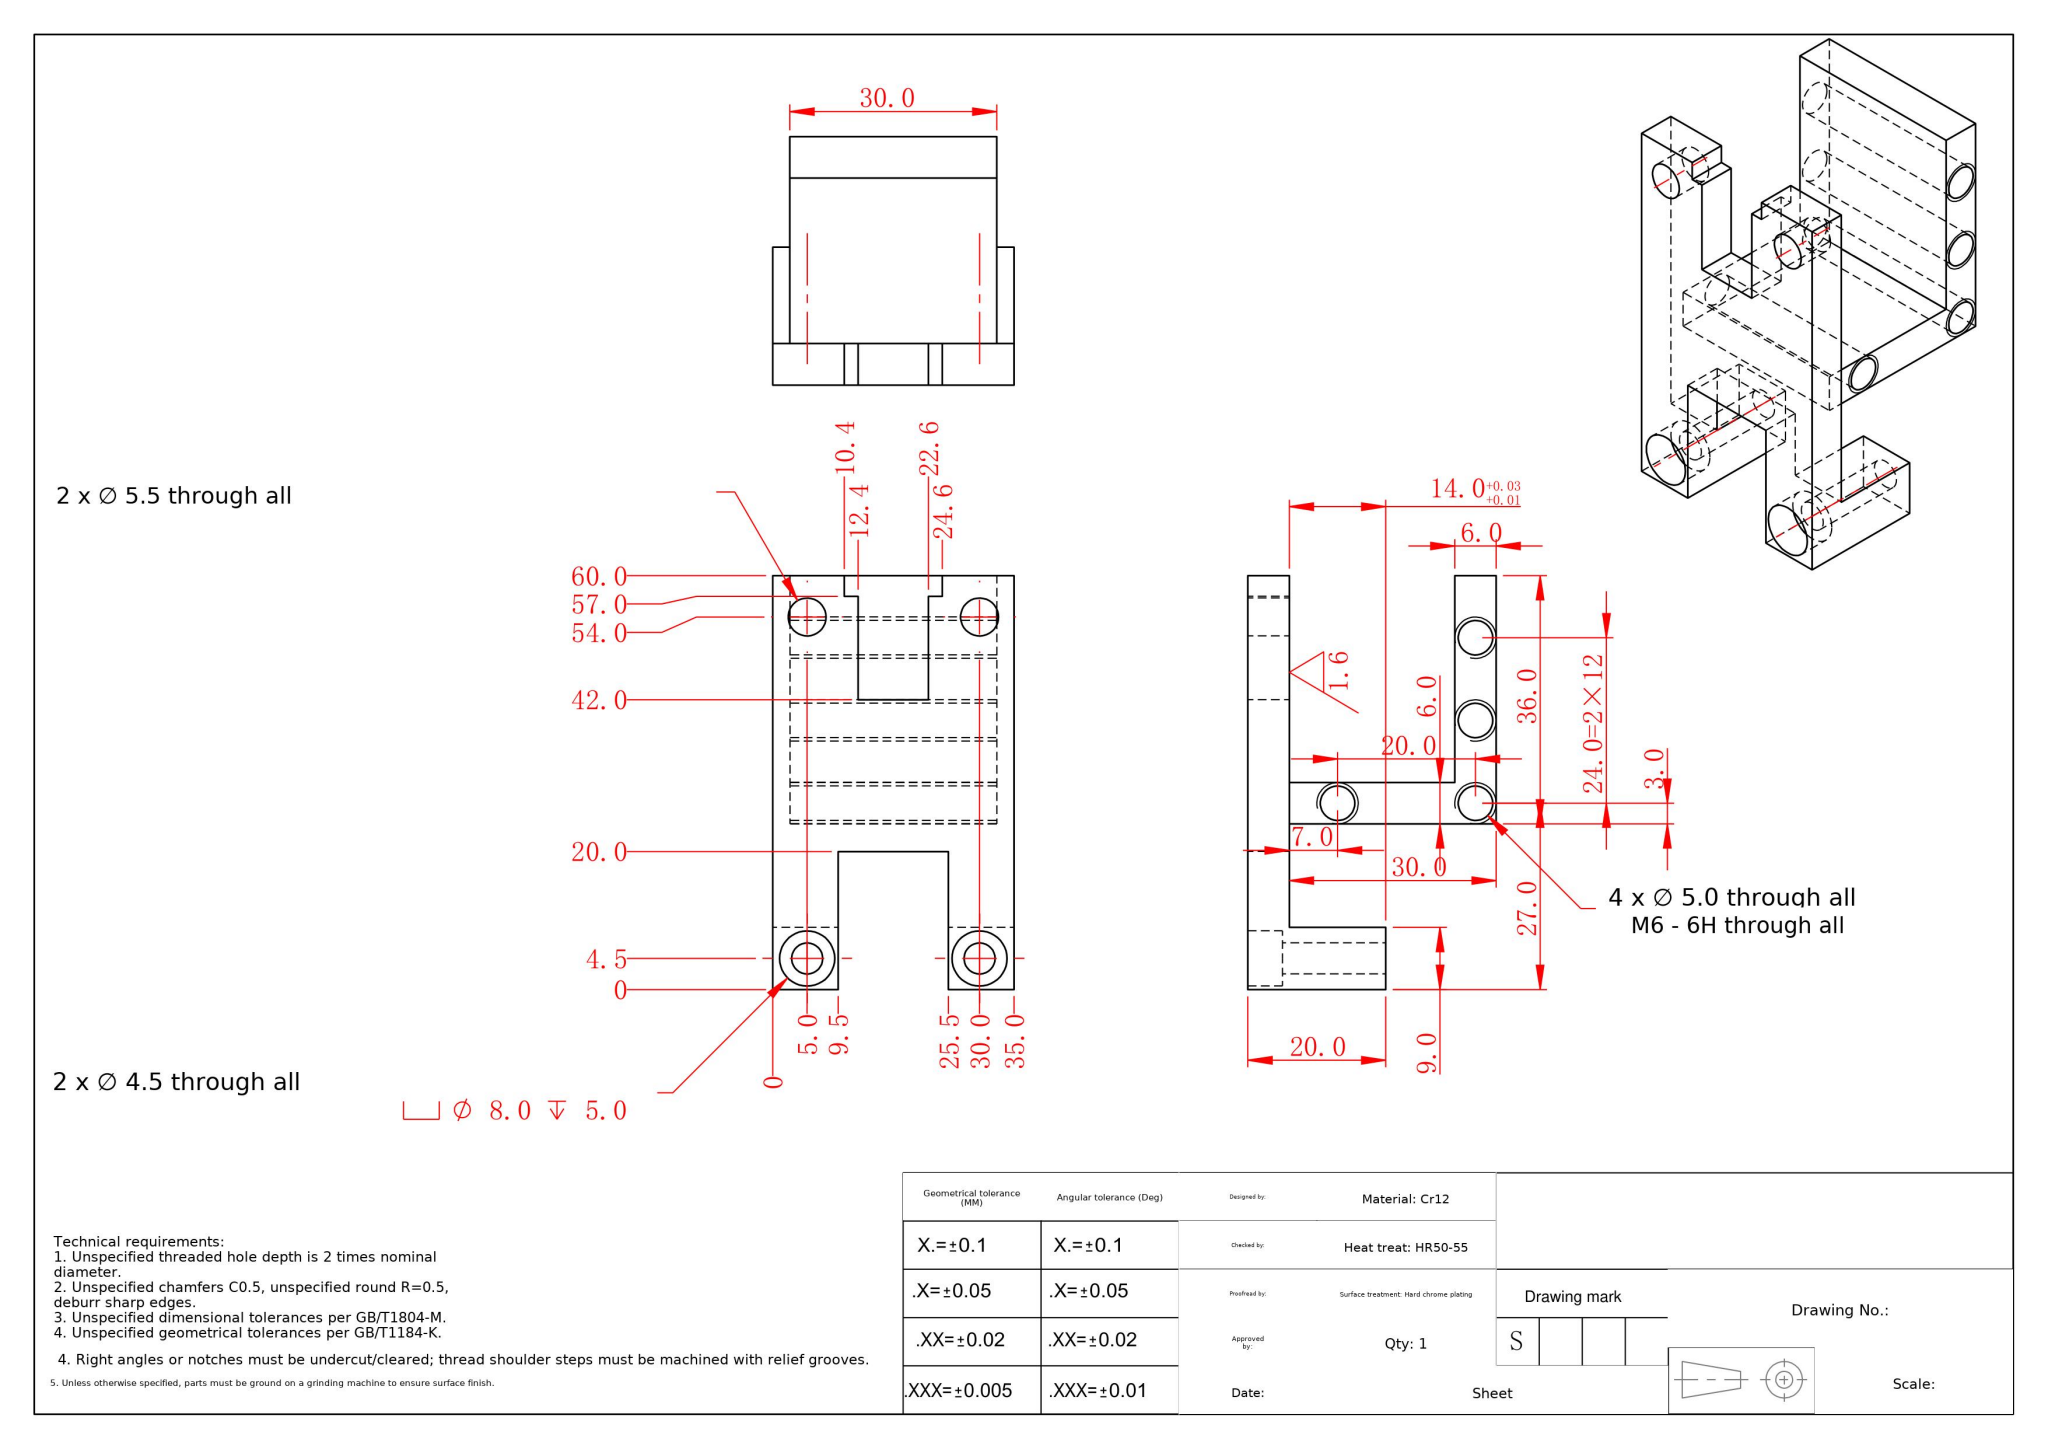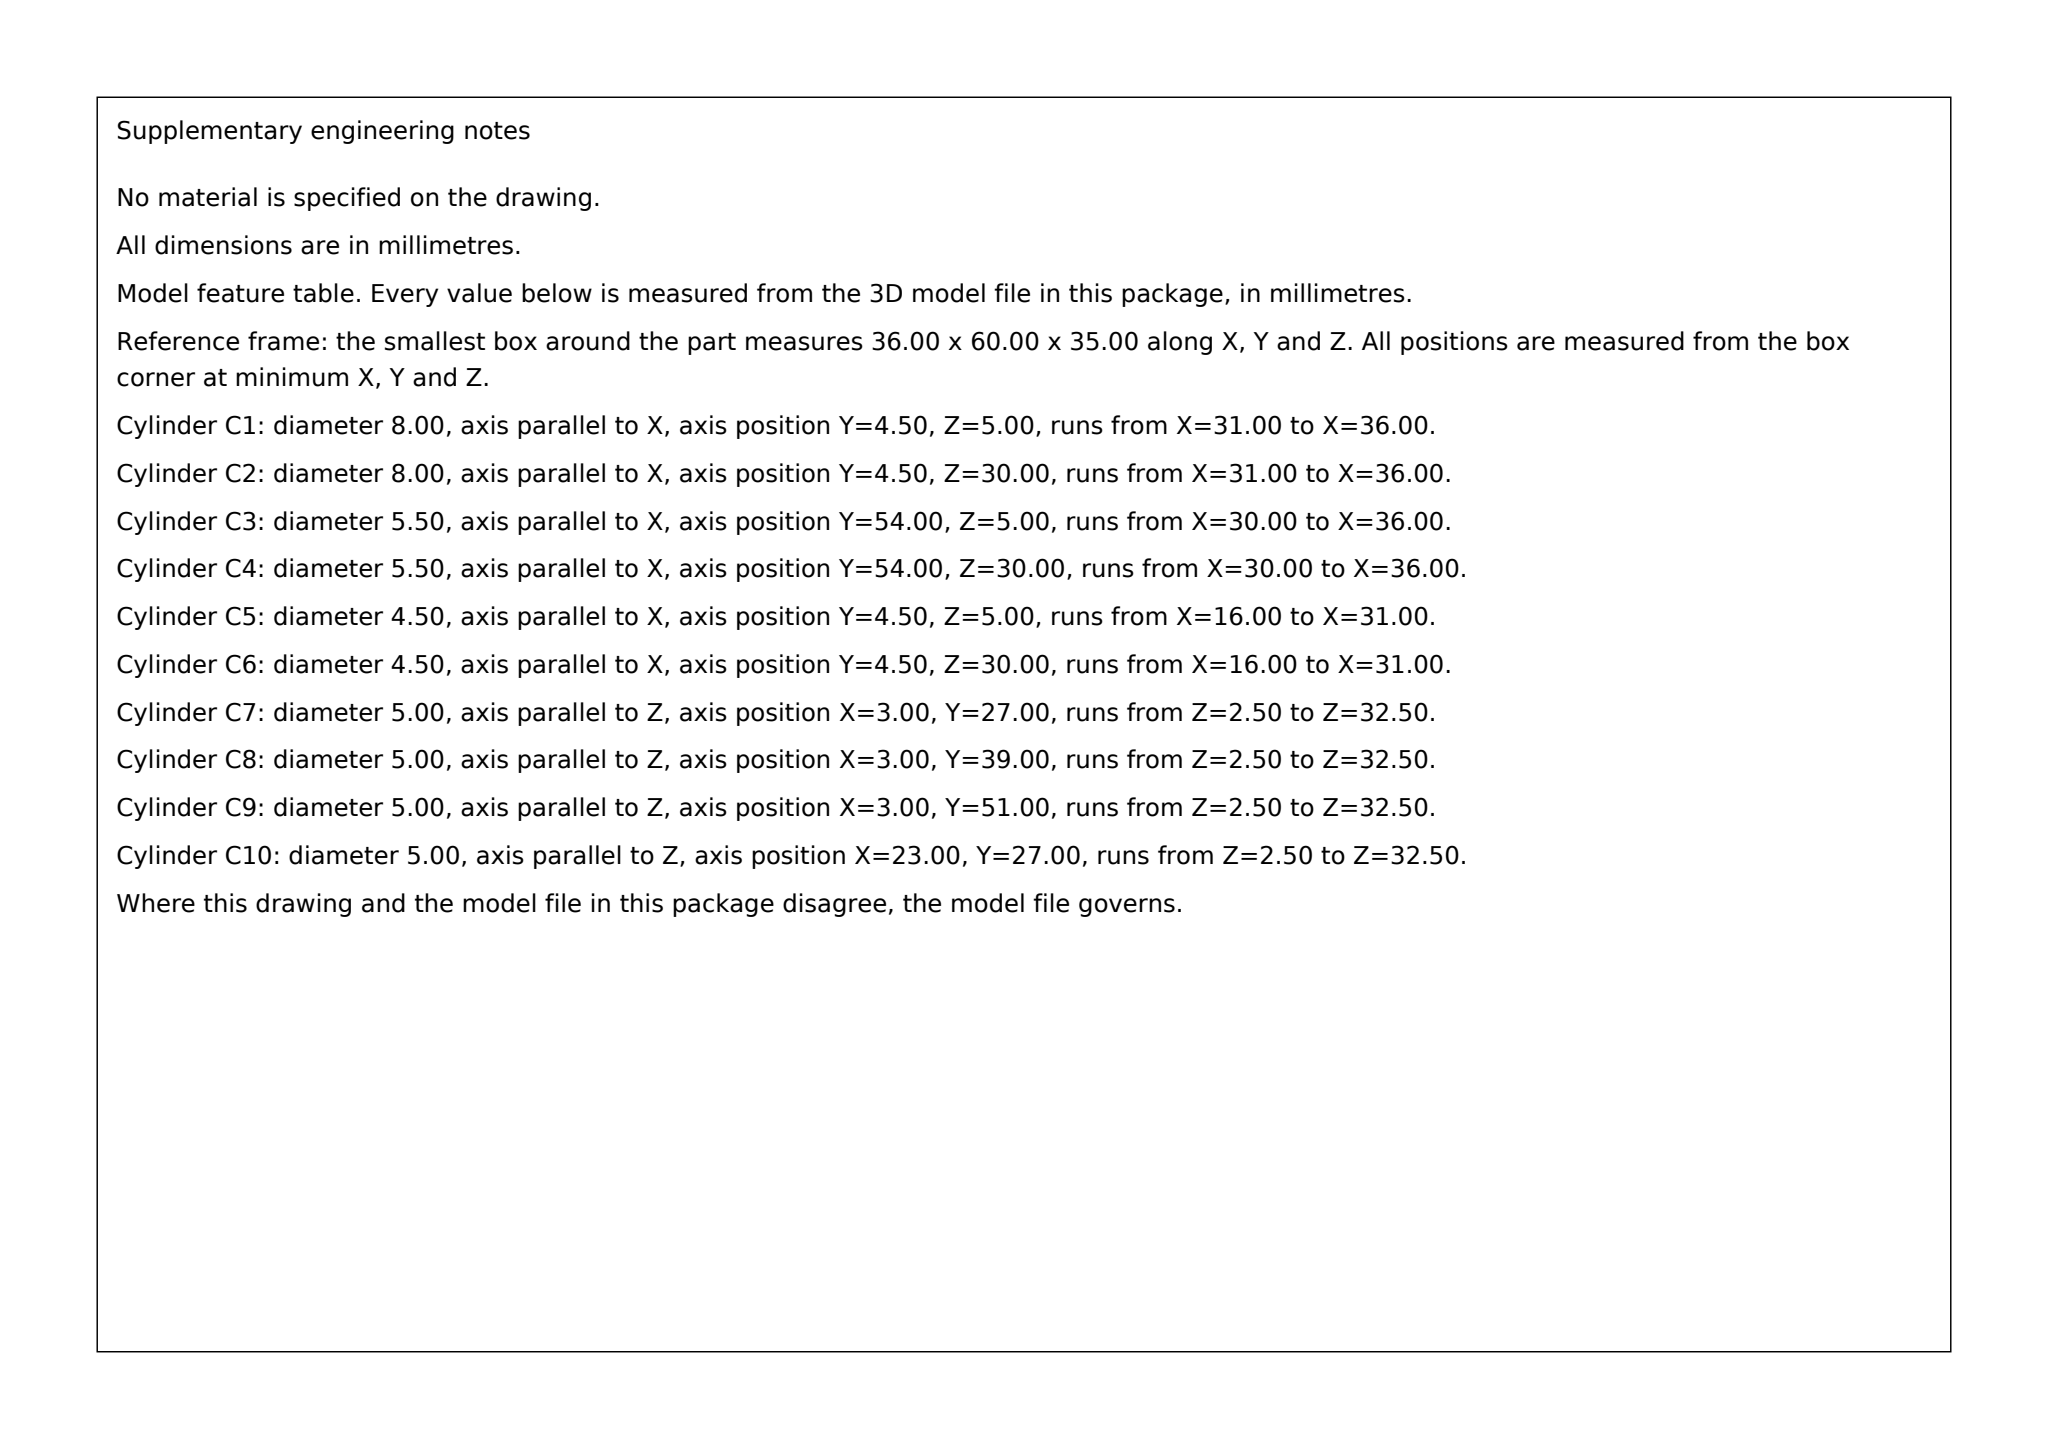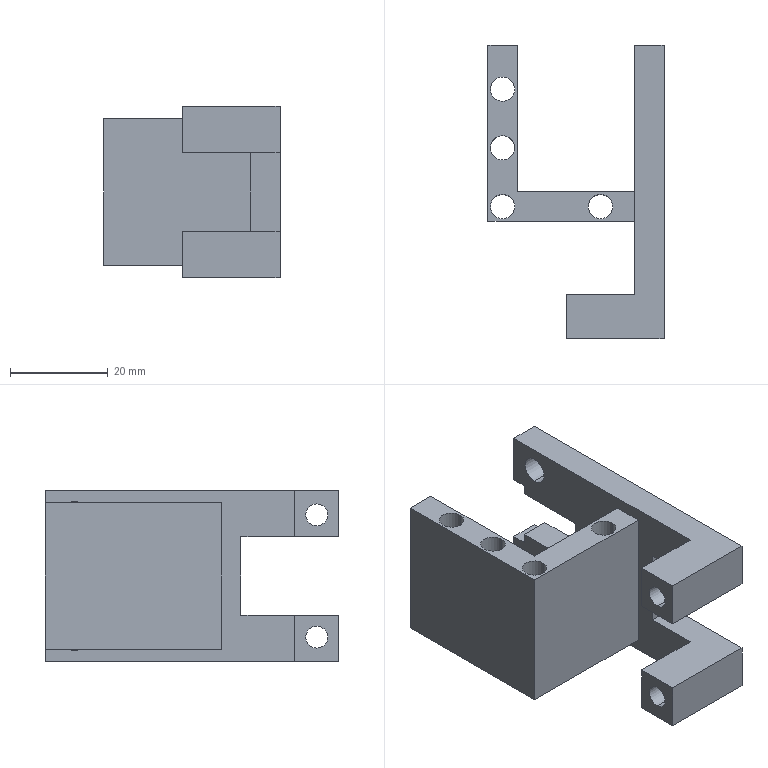Part | SolidWorks | mm | 1 solid | 51 faces | box 36 x 60 x 35 mm | volume 19079 mm3 | plane 31 | cylinder 20 | commonest cylinder face diameters 5 x8 8 x4 4.5 x4 5.5 x4
build123d program:
from build123d import *

# Parameters (mm, degrees)
SKETCH1_W                                       = 6
SKETCH1_H                                       = 60
BOSS_EXTRUDE1_DEPTH                             = 17.5
SKETCH3_W                                       = 10.2
SKETCH3_H                                       = 18
CUT_EXTRUDE2_DEPTH                              = 63.787
F_5_5_5_5_DIAMETER_HOLE2_D                      = 5.5
SKETCH7_W                                       = 9.5
SKETCH7_H                                       = 9
BOSS_EXTRUDE2_DEPTH                             = 14
SKETCH8_W                                       = 6
SKETCH8_H                                       = 16
CUT_EXTRUDE3_DEPTH                              = 20
M4_HEX_SOCKET_HEAD_CAP_SCREW_CBORE1_D           = 4.5
M4_HEX_SOCKET_HEAD_CAP_SCREW_CBORE1_CBORE_D     = 8
M4_HEX_SOCKET_HEAD_CAP_SCREW_CBORE1_CBORE_DEPTH = 5
CUT_EXTRUDE4_REACH                              = 67.622
SKETCH11_W                                      = 2
SKETCH11_H                                      = 3
BOSS_EXTRUDE3_DEPTH                             = 15
M6_TAPPED_HOLE1_D                               = 5


with BuildPart() as part:
    # Sketch1 → Boss-Extrude1 (new, symmetric)
    with BuildSketch(Plane.XY):
        with Locations((0, -30)):
            Rectangle(SKETCH1_W, SKETCH1_H)
    extrude(amount=BOSS_EXTRUDE1_DEPTH, both=True)

    # Sketch3 → Cut-Extrude2 (cut, through all)
    with BuildSketch(Plane(origin=(3, 0, 0), x_dir=(0, 0, -1), z_dir=(1, 0, 0))):
        with Locations((0, -9)):
            Rectangle(SKETCH3_W, SKETCH3_H)
    extrude(amount=-CUT_EXTRUDE2_DEPTH, mode=Mode.SUBTRACT)

    # 5.5 _5.5_ Diameter Hole2 (through all)
    with Locations(Plane(origin=(3, 0, 0), x_dir=(0, 0, -1), z_dir=(1, 0, 0))):
        with Locations((-12.5, -6), (12.5, -6)):
            Hole(F_5_5_5_5_DIAMETER_HOLE2_D / 2)

    # Sketch7 → Boss-Extrude2 (add)
    with BuildSketch(Plane.ZY.offset(3)):
        with Locations((12.75, -55.5)):
            Rectangle(SKETCH7_W, SKETCH7_H)
        with Locations((-12.75, -55.5)):
            Rectangle(SKETCH7_W, SKETCH7_H)
    extrude(amount=BOSS_EXTRUDE2_DEPTH)

    # Sketch8 → Cut-Extrude3 (cut)
    with BuildSketch(Plane.XZ.offset(60)):
        Rectangle(SKETCH8_W, SKETCH8_H)
    extrude(amount=-CUT_EXTRUDE3_DEPTH, mode=Mode.SUBTRACT)

    # M4 Hex Socket Head Cap Screw CBORE1 (through all)
    with Locations(Plane(origin=(3, 0, 0), x_dir=(0, 0, -1), z_dir=(1, 0, 0))):
        with Locations((-12.5, -55.5), (12.5, -55.5)):
            CounterBoreHole(M4_HEX_SOCKET_HEAD_CAP_SCREW_CBORE1_D / 2, M4_HEX_SOCKET_HEAD_CAP_SCREW_CBORE1_CBORE_D / 2, M4_HEX_SOCKET_HEAD_CAP_SCREW_CBORE1_CBORE_DEPTH)

    # Sketch11 → Cut-Extrude4 (cut, up to next)
    with BuildSketch(Plane(origin=(3, 0, 0), x_dir=(0, 0, -1), z_dir=(1, 0, 0)), mode=Mode.PRIVATE) as cut_extrude4_sk1:
        with Locations((-6.1, -1.5)):
            Rectangle(SKETCH11_W, SKETCH11_H)
    cut_extrude4_tool1 = extrude(cut_extrude4_sk1.sketch, amount=-CUT_EXTRUDE4_REACH, mode=Mode.PRIVATE) & part.part
    # Sketch11 → Cut-Extrude4 (cut, up to next)
    with BuildSketch(Plane(origin=(3, 0, 0), x_dir=(0, 0, -1), z_dir=(1, 0, 0)), mode=Mode.PRIVATE) as cut_extrude4_sk2:
        with Locations((6.1, -1.5)):
            Rectangle(SKETCH11_W, SKETCH11_H)
    cut_extrude4_tool2 = extrude(cut_extrude4_sk2.sketch, amount=-CUT_EXTRUDE4_REACH, mode=Mode.PRIVATE) & part.part
    add(cut_extrude4_tool1.solids().sort_by_distance((3, -1.5, 6.1))[0], mode=Mode.SUBTRACT)
    add(cut_extrude4_tool2.solids().sort_by_distance((3, -1.5, -6.1))[0], mode=Mode.SUBTRACT)

    # Sketch12 → Boss-Extrude3 (add, symmetric)
    with BuildSketch(Plane.XY):
        Polygon((-3, -36), (-33, -36), (-33, 0), (-27, 0), (-27, -30), (-3, -30), align=None)
    extrude(amount=BOSS_EXTRUDE3_DEPTH, both=True)

    # M6 Tapped Hole1 (through all)
    with Locations(Plane(origin=(0, 0, -15), x_dir=(-1, 0, 0), z_dir=(0, 0, -1))):
        with Locations((30, -9), (30, -21), (30, -33), (10, -33)):
            Hole(M6_TAPPED_HOLE1_D / 2)


solid = part.part